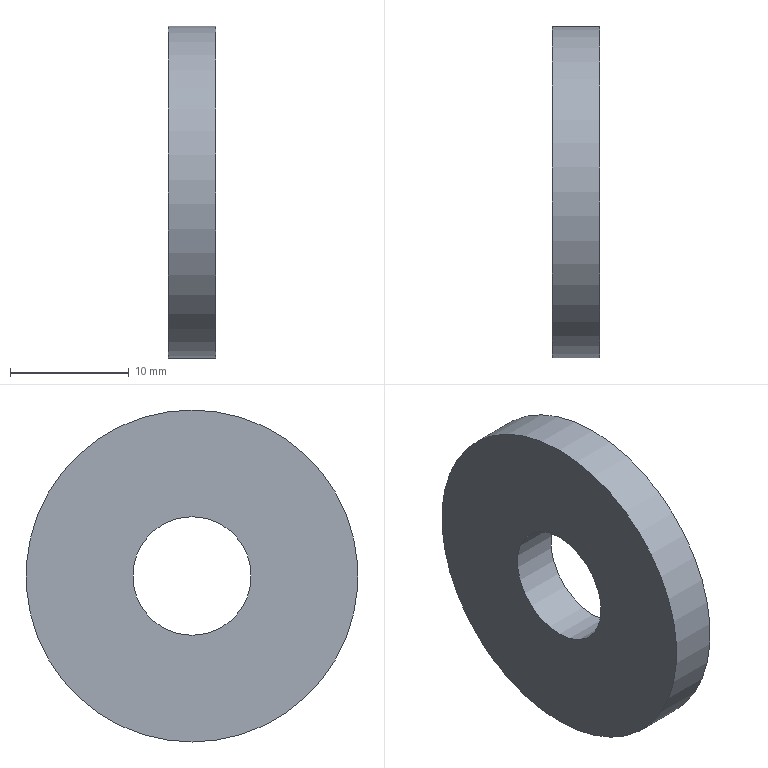Component | NX | SUPPORT_RING | 1 solid | 4 faces | box 4 x 28 x 28 mm | volume 2149 mm3 | cylinder 2 | plane 2 | commonest cylinder face diameters 28 x1 10 x1
STEP:
#1=CARTESIAN_POINT('',(0.,0.,0.));
#2=DIRECTION('',(0.,0.,1.));
#3=DIRECTION('',(1.,0.,0.));
#4=AXIS2_PLACEMENT_3D('',#1,#2,#3);
#5=CARTESIAN_POINT('',(-39.,-0.,50.5));
#6=VERTEX_POINT('',#5);
#7=CARTESIAN_POINT('',(-39.,-0.,36.5));
#8=DIRECTION('',(-1.,0.,0.));
#9=DIRECTION('',(0.,0.,1.));
#10=AXIS2_PLACEMENT_3D('',#7,#8,#9);
#11=CIRCLE('',#10,14.);
#12=CARTESIAN_POINT('',(-39.,-0.,36.5));
#13=DIRECTION('',(1.,0.,0.));
#14=DIRECTION('',(0.,0.,-1.));
#15=AXIS2_PLACEMENT_3D('',#12,#13,#14);
#16=CYLINDRICAL_SURFACE('',#15,14.);
#17=CARTESIAN_POINT('',(9.425,0.));
#18=DIRECTION('',(-1.,0.));
#19=VECTOR('',#18,1.);
#20=LINE('',#17,#19);
#21=(GEOMETRIC_REPRESENTATION_CONTEXT(2)PARAMETRIC_REPRESENTATION_CONTEXT()REPRESENTATION_CONTEXT('',''));
#22=DEFINITIONAL_REPRESENTATION('',(#20),#21);
#23=PCURVE('',#16,#22);
#24=CARTESIAN_POINT('',(-39.,-0.,36.5));
#25=DIRECTION('',(-1.,0.,0.));
#26=DIRECTION('',(0.,0.,1.));
#27=AXIS2_PLACEMENT_3D('',#24,#25,#26);
#28=PLANE('',#27);
#29=CARTESIAN_POINT('',(0.,0.));
#30=DIRECTION('',(1.,0.));
#31=AXIS2_PLACEMENT_2D('',#29,#30);
#32=CIRCLE('',#31,14.);
#33=(GEOMETRIC_REPRESENTATION_CONTEXT(2)PARAMETRIC_REPRESENTATION_CONTEXT()REPRESENTATION_CONTEXT('',''));
#34=DEFINITIONAL_REPRESENTATION('',(#32),#33);
#35=PCURVE('',#28,#34);
#36=SURFACE_CURVE('',#11,(#23,#35),.PCURVE_S1.);
#37=EDGE_CURVE('',#6,#6,#36,.T.);
#38=ORIENTED_EDGE('',*,*,#37,.F.);
#39=CARTESIAN_POINT('',(-35.,-0.,50.5));
#40=VERTEX_POINT('',#39);
#41=CARTESIAN_POINT('',(-39.,-0.,50.5));
#42=CARTESIAN_POINT('',(-35.,-0.,50.5));
#43=B_SPLINE_CURVE_WITH_KNOTS('',1,(#41,#42),.UNSPECIFIED.,.F.,.F.,(2,2),(0.,4.),.PIECEWISE_BEZIER_KNOTS.);
#44=CARTESIAN_POINT('',(9.425,0.));
#45=DIRECTION('',(0.,1.));
#46=VECTOR('',#45,1.);
#47=LINE('',#44,#46);
#48=(GEOMETRIC_REPRESENTATION_CONTEXT(2)PARAMETRIC_REPRESENTATION_CONTEXT()REPRESENTATION_CONTEXT('',''));
#49=DEFINITIONAL_REPRESENTATION('',(#47),#48);
#50=PCURVE('',#16,#49);
#51=CARTESIAN_POINT('',(3.142,0.));
#52=DIRECTION('',(0.,1.));
#53=VECTOR('',#52,1.);
#54=LINE('',#51,#53);
#55=(GEOMETRIC_REPRESENTATION_CONTEXT(2)PARAMETRIC_REPRESENTATION_CONTEXT()REPRESENTATION_CONTEXT('',''));
#56=DEFINITIONAL_REPRESENTATION('',(#54),#55);
#57=PCURVE('',#16,#56);
#58=SEAM_CURVE('',#43,(#50,#57),.PCURVE_S1.);
#59=EDGE_CURVE('',#6,#40,#58,.T.);
#60=ORIENTED_EDGE('',*,*,#59,.T.);
#61=CARTESIAN_POINT('',(-35.,-0.,36.5));
#62=DIRECTION('',(-1.,0.,0.));
#63=DIRECTION('',(0.,0.,1.));
#64=AXIS2_PLACEMENT_3D('',#61,#62,#63);
#65=CIRCLE('',#64,14.);
#66=CARTESIAN_POINT('',(9.425,4.));
#67=DIRECTION('',(-1.,0.));
#68=VECTOR('',#67,1.);
#69=LINE('',#66,#68);
#70=(GEOMETRIC_REPRESENTATION_CONTEXT(2)PARAMETRIC_REPRESENTATION_CONTEXT()REPRESENTATION_CONTEXT('',''));
#71=DEFINITIONAL_REPRESENTATION('',(#69),#70);
#72=PCURVE('',#16,#71);
#73=CARTESIAN_POINT('',(-35.,-0.,36.5));
#74=DIRECTION('',(-1.,0.,0.));
#75=DIRECTION('',(0.,0.,1.));
#76=AXIS2_PLACEMENT_3D('',#73,#74,#75);
#77=PLANE('',#76);
#78=CARTESIAN_POINT('',(0.,0.));
#79=DIRECTION('',(1.,0.));
#80=AXIS2_PLACEMENT_2D('',#78,#79);
#81=CIRCLE('',#80,14.);
#82=(GEOMETRIC_REPRESENTATION_CONTEXT(2)PARAMETRIC_REPRESENTATION_CONTEXT()REPRESENTATION_CONTEXT('',''));
#83=DEFINITIONAL_REPRESENTATION('',(#81),#82);
#84=PCURVE('',#77,#83);
#85=SURFACE_CURVE('',#65,(#72,#84),.PCURVE_S1.);
#86=EDGE_CURVE('',#40,#40,#85,.T.);
#87=ORIENTED_EDGE('',*,*,#86,.T.);
#88=ORIENTED_EDGE('',*,*,#59,.F.);
#89=EDGE_LOOP('',(#38,#60,#87,#88));
#90=FACE_BOUND('',#89,.T.);
#91=ADVANCED_FACE('',(#90),#16,.T.);
#92=CARTESIAN_POINT('',(-39.,-0.,41.5));
#93=VERTEX_POINT('',#92);
#94=CARTESIAN_POINT('',(-39.,-0.,36.5));
#95=DIRECTION('',(-1.,0.,0.));
#96=DIRECTION('',(0.,0.,1.));
#97=AXIS2_PLACEMENT_3D('',#94,#95,#96);
#98=CIRCLE('',#97,5.);
#99=CARTESIAN_POINT('',(-39.,-0.,36.5));
#100=DIRECTION('',(1.,0.,0.));
#101=DIRECTION('',(0.,0.,-1.));
#102=AXIS2_PLACEMENT_3D('',#99,#100,#101);
#103=CYLINDRICAL_SURFACE('',#102,5.);
#104=CARTESIAN_POINT('',(9.425,0.));
#105=DIRECTION('',(-1.,0.));
#106=VECTOR('',#105,1.);
#107=LINE('',#104,#106);
#108=(GEOMETRIC_REPRESENTATION_CONTEXT(2)PARAMETRIC_REPRESENTATION_CONTEXT()REPRESENTATION_CONTEXT('',''));
#109=DEFINITIONAL_REPRESENTATION('',(#107),#108);
#110=PCURVE('',#103,#109);
#111=CARTESIAN_POINT('',(0.,0.));
#112=DIRECTION('',(1.,0.));
#113=AXIS2_PLACEMENT_2D('',#111,#112);
#114=CIRCLE('',#113,5.);
#115=(GEOMETRIC_REPRESENTATION_CONTEXT(2)PARAMETRIC_REPRESENTATION_CONTEXT()REPRESENTATION_CONTEXT('',''));
#116=DEFINITIONAL_REPRESENTATION('',(#114),#115);
#117=PCURVE('',#28,#116);
#118=SURFACE_CURVE('',#98,(#110,#117),.PCURVE_S1.);
#119=EDGE_CURVE('',#93,#93,#118,.T.);
#120=ORIENTED_EDGE('',*,*,#119,.F.);
#121=CARTESIAN_POINT('',(-35.,-0.,41.5));
#122=VERTEX_POINT('',#121);
#123=CARTESIAN_POINT('',(-39.,-0.,41.5));
#124=CARTESIAN_POINT('',(-35.,-0.,41.5));
#125=B_SPLINE_CURVE_WITH_KNOTS('',1,(#123,#124),.UNSPECIFIED.,.F.,.F.,(2,2),(0.,4.),.PIECEWISE_BEZIER_KNOTS.);
#126=CARTESIAN_POINT('',(9.425,0.));
#127=DIRECTION('',(0.,1.));
#128=VECTOR('',#127,1.);
#129=LINE('',#126,#128);
#130=(GEOMETRIC_REPRESENTATION_CONTEXT(2)PARAMETRIC_REPRESENTATION_CONTEXT()REPRESENTATION_CONTEXT('',''));
#131=DEFINITIONAL_REPRESENTATION('',(#129),#130);
#132=PCURVE('',#103,#131);
#133=CARTESIAN_POINT('',(3.142,0.));
#134=DIRECTION('',(0.,1.));
#135=VECTOR('',#134,1.);
#136=LINE('',#133,#135);
#137=(GEOMETRIC_REPRESENTATION_CONTEXT(2)PARAMETRIC_REPRESENTATION_CONTEXT()REPRESENTATION_CONTEXT('',''));
#138=DEFINITIONAL_REPRESENTATION('',(#136),#137);
#139=PCURVE('',#103,#138);
#140=SEAM_CURVE('',#125,(#132,#139),.PCURVE_S1.);
#141=EDGE_CURVE('',#93,#122,#140,.T.);
#142=ORIENTED_EDGE('',*,*,#141,.T.);
#143=CARTESIAN_POINT('',(-35.,-0.,36.5));
#144=DIRECTION('',(-1.,0.,0.));
#145=DIRECTION('',(0.,0.,1.));
#146=AXIS2_PLACEMENT_3D('',#143,#144,#145);
#147=CIRCLE('',#146,5.);
#148=CARTESIAN_POINT('',(9.425,4.));
#149=DIRECTION('',(-1.,0.));
#150=VECTOR('',#149,1.);
#151=LINE('',#148,#150);
#152=(GEOMETRIC_REPRESENTATION_CONTEXT(2)PARAMETRIC_REPRESENTATION_CONTEXT()REPRESENTATION_CONTEXT('',''));
#153=DEFINITIONAL_REPRESENTATION('',(#151),#152);
#154=PCURVE('',#103,#153);
#155=CARTESIAN_POINT('',(0.,0.));
#156=DIRECTION('',(1.,0.));
#157=AXIS2_PLACEMENT_2D('',#155,#156);
#158=CIRCLE('',#157,5.);
#159=(GEOMETRIC_REPRESENTATION_CONTEXT(2)PARAMETRIC_REPRESENTATION_CONTEXT()REPRESENTATION_CONTEXT('',''));
#160=DEFINITIONAL_REPRESENTATION('',(#158),#159);
#161=PCURVE('',#77,#160);
#162=SURFACE_CURVE('',#147,(#154,#161),.PCURVE_S1.);
#163=EDGE_CURVE('',#122,#122,#162,.T.);
#164=ORIENTED_EDGE('',*,*,#163,.T.);
#165=ORIENTED_EDGE('',*,*,#141,.F.);
#166=EDGE_LOOP('',(#120,#142,#164,#165));
#167=FACE_BOUND('',#166,.F.);
#168=ADVANCED_FACE('',(#167),#103,.F.);
#169=ORIENTED_EDGE('',*,*,#37,.T.);
#170=EDGE_LOOP('',(#169));
#171=FACE_BOUND('',#170,.T.);
#172=ORIENTED_EDGE('',*,*,#119,.F.);
#173=EDGE_LOOP('',(#172));
#174=FACE_BOUND('',#173,.T.);
#175=ADVANCED_FACE('',(#171,#174),#28,.T.);
#176=ORIENTED_EDGE('',*,*,#86,.F.);
#177=EDGE_LOOP('',(#176));
#178=FACE_BOUND('',#177,.T.);
#179=ORIENTED_EDGE('',*,*,#163,.T.);
#180=EDGE_LOOP('',(#179));
#181=FACE_BOUND('',#180,.T.);
#182=ADVANCED_FACE('',(#178,#181),#77,.F.);
#183=CLOSED_SHELL('',(#91,#168,#175,#182));
#184=MANIFOLD_SOLID_BREP('',#183);
#185=(LENGTH_UNIT()NAMED_UNIT(*)SI_UNIT(.MILLI.,.METRE.));
#186=UNCERTAINTY_MEASURE_WITH_UNIT(LENGTH_MEASURE(0.00001),#185,'','');
#187=(NAMED_UNIT(*)PLANE_ANGLE_UNIT()SI_UNIT($,.RADIAN.));
#188=(NAMED_UNIT(*)SI_UNIT($,.STERADIAN.)SOLID_ANGLE_UNIT());
#189=(GEOMETRIC_REPRESENTATION_CONTEXT(3)GLOBAL_UNCERTAINTY_ASSIGNED_CONTEXT((#186))GLOBAL_UNIT_ASSIGNED_CONTEXT((#185,#187,#188))REPRESENTATION_CONTEXT('',''));
#190=ADVANCED_BREP_SHAPE_REPRESENTATION('',(#4,#184),#189);